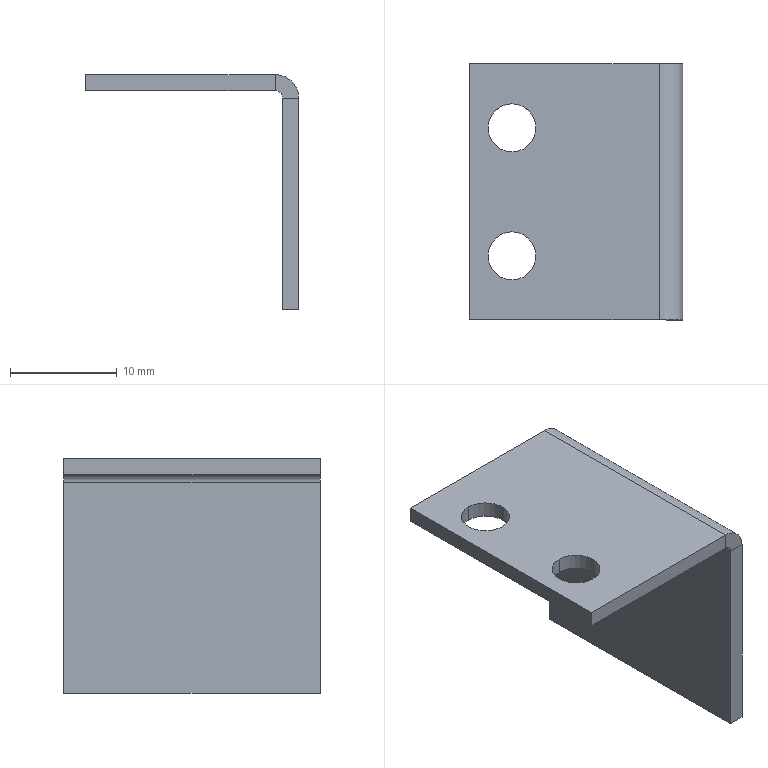Component | SolidWorks | 17081801-804-017B-1 | 1 solid | 18 faces | box 20 x 24 x 22 mm | volume 1388 mm3 | plane 12 | cylinder 6 | commonest cylinder face diameters 4.5 x4 4.4 x1 1.4 x1 | material 1.5mm304 Stainless Steel
STEP:
#1=COLOUR_RGB('',0.7922,0.8196,0.9333);
#2=FILL_AREA_STYLE_COLOUR('',#1);
#3=FILL_AREA_STYLE('',(#2));
#4=SURFACE_STYLE_FILL_AREA(#3);
#5=SURFACE_SIDE_STYLE('',(#4));
#6=SURFACE_STYLE_USAGE(.BOTH.,#5);
#7=PRESENTATION_STYLE_ASSIGNMENT((#6));
#8=CARTESIAN_POINT('',(1.043,83.234,5.335));
#9=VERTEX_POINT('',#8);
#10=CARTESIAN_POINT('',(1.043,83.057,5.335));
#11=VERTEX_POINT('',#10);
#12=CARTESIAN_POINT('',(1.043,83.146,5.335));
#13=DIRECTION('',(0.,-0.,1.));
#14=DIRECTION('',(-0.,-1.,0.));
#15=AXIS2_PLACEMENT_3D('',#12,#13,#14);
#16=CIRCLE('',#15,0.08858);
#17=EDGE_CURVE('',#9,#11,#16,.T.);
#18=ORIENTED_EDGE('',*,*,#17,.T.);
#19=CARTESIAN_POINT('',(1.043,83.057,5.276));
#20=VERTEX_POINT('',#19);
#21=CARTESIAN_POINT('',(1.043,83.057,5.276));
#22=DIRECTION('',(-0.,0.,-1.));
#23=VECTOR('',#22,39.37);
#24=LINE('',#21,#23);
#25=EDGE_CURVE('',#11,#20,#24,.T.);
#26=ORIENTED_EDGE('',*,*,#25,.T.);
#27=CARTESIAN_POINT('',(1.043,83.234,5.276));
#28=VERTEX_POINT('',#27);
#29=CARTESIAN_POINT('',(1.043,83.146,5.276));
#30=DIRECTION('',(-0.,0.,-1.));
#31=DIRECTION('',(0.,1.,0.));
#32=AXIS2_PLACEMENT_3D('',#29,#30,#31);
#33=CIRCLE('',#32,0.08858);
#34=EDGE_CURVE('',#20,#28,#33,.T.);
#35=ORIENTED_EDGE('',*,*,#34,.T.);
#36=CARTESIAN_POINT('',(1.043,83.234,5.276));
#37=DIRECTION('',(-0.,0.,-1.));
#38=VECTOR('',#37,39.37);
#39=LINE('',#36,#38);
#40=EDGE_CURVE('',#9,#28,#39,.T.);
#41=ORIENTED_EDGE('',*,*,#40,.F.);
#42=EDGE_LOOP('',(#18,#26,#35,#41));
#43=FACE_OUTER_BOUND('',#42,.T.);
#44=CARTESIAN_POINT('',(1.043,83.146,5.276));
#45=DIRECTION('',(-0.,0.,-1.));
#46=DIRECTION('',(0.,1.,0.));
#47=AXIS2_PLACEMENT_3D('',#44,#45,#46);
#48=CYLINDRICAL_SURFACE('',#47,0.08858);
#49=ADVANCED_FACE('',(#43),#48,.F.);
#50=CARTESIAN_POINT('',(1.043,83.707,5.335));
#51=VERTEX_POINT('',#50);
#52=CARTESIAN_POINT('',(1.043,83.53,5.335));
#53=VERTEX_POINT('',#52);
#54=CARTESIAN_POINT('',(1.043,83.618,5.335));
#55=DIRECTION('',(0.,-0.,1.));
#56=DIRECTION('',(-0.,-1.,0.));
#57=AXIS2_PLACEMENT_3D('',#54,#55,#56);
#58=CIRCLE('',#57,0.08858);
#59=EDGE_CURVE('',#51,#53,#58,.T.);
#60=ORIENTED_EDGE('',*,*,#59,.T.);
#61=CARTESIAN_POINT('',(1.043,83.53,5.276));
#62=VERTEX_POINT('',#61);
#63=CARTESIAN_POINT('',(1.043,83.53,5.276));
#64=DIRECTION('',(-0.,0.,-1.));
#65=VECTOR('',#64,39.37);
#66=LINE('',#63,#65);
#67=EDGE_CURVE('',#53,#62,#66,.T.);
#68=ORIENTED_EDGE('',*,*,#67,.T.);
#69=CARTESIAN_POINT('',(1.043,83.707,5.276));
#70=VERTEX_POINT('',#69);
#71=CARTESIAN_POINT('',(1.043,83.618,5.276));
#72=DIRECTION('',(-0.,0.,-1.));
#73=DIRECTION('',(0.,1.,0.));
#74=AXIS2_PLACEMENT_3D('',#71,#72,#73);
#75=CIRCLE('',#74,0.08858);
#76=EDGE_CURVE('',#62,#70,#75,.T.);
#77=ORIENTED_EDGE('',*,*,#76,.T.);
#78=CARTESIAN_POINT('',(1.043,83.707,5.276));
#79=DIRECTION('',(-0.,0.,-1.));
#80=VECTOR('',#79,39.37);
#81=LINE('',#78,#80);
#82=EDGE_CURVE('',#51,#70,#81,.T.);
#83=ORIENTED_EDGE('',*,*,#82,.F.);
#84=EDGE_LOOP('',(#60,#68,#77,#83));
#85=FACE_OUTER_BOUND('',#84,.T.);
#86=CARTESIAN_POINT('',(1.043,83.618,5.276));
#87=DIRECTION('',(-0.,0.,-1.));
#88=DIRECTION('',(0.,1.,0.));
#89=AXIS2_PLACEMENT_3D('',#86,#87,#88);
#90=CYLINDRICAL_SURFACE('',#89,0.08858);
#91=ADVANCED_FACE('',(#85),#90,.F.);
#92=CARTESIAN_POINT('',(1.673,82.909,5.248));
#93=VERTEX_POINT('',#92);
#94=CARTESIAN_POINT('',(1.614,82.909,5.248));
#95=VERTEX_POINT('',#94);
#96=CARTESIAN_POINT('',(1.673,82.909,5.248));
#97=DIRECTION('',(-1.,0.,0.));
#98=VECTOR('',#97,39.37);
#99=LINE('',#96,#98);
#100=EDGE_CURVE('',#93,#95,#99,.T.);
#101=ORIENTED_EDGE('',*,*,#100,.F.);
#102=CARTESIAN_POINT('',(1.587,82.909,5.335));
#103=VERTEX_POINT('',#102);
#104=CARTESIAN_POINT('',(1.587,82.909,5.248));
#105=DIRECTION('',(0.,1.,0.));
#106=DIRECTION('',(1.,0.,0.));
#107=AXIS2_PLACEMENT_3D('',#104,#105,#106);
#108=CIRCLE('',#107,0.08661);
#109=EDGE_CURVE('',#103,#93,#108,.T.);
#110=ORIENTED_EDGE('',*,*,#109,.F.);
#111=CARTESIAN_POINT('',(1.587,82.909,5.276));
#112=VERTEX_POINT('',#111);
#113=CARTESIAN_POINT('',(1.587,82.909,5.276));
#114=DIRECTION('',(-0.,-0.,1.));
#115=VECTOR('',#114,39.37);
#116=LINE('',#113,#115);
#117=EDGE_CURVE('',#112,#103,#116,.T.);
#118=ORIENTED_EDGE('',*,*,#117,.F.);
#119=CARTESIAN_POINT('',(1.587,82.909,5.248));
#120=DIRECTION('',(0.,1.,0.));
#121=DIRECTION('',(1.,0.,0.));
#122=AXIS2_PLACEMENT_3D('',#119,#120,#121);
#123=CIRCLE('',#122,0.02756);
#124=EDGE_CURVE('',#112,#95,#123,.T.);
#125=ORIENTED_EDGE('',*,*,#124,.T.);
#126=EDGE_LOOP('',(#101,#110,#118,#125));
#127=FACE_OUTER_BOUND('',#126,.T.);
#128=CARTESIAN_POINT('',(1.673,82.909,5.248));
#129=DIRECTION('',(-0.,-1.,-0.));
#130=DIRECTION('',(1.,-0.,-0.));
#131=AXIS2_PLACEMENT_3D('',#128,#129,#130);
#132=PLANE('',#131);
#133=ADVANCED_FACE('',(#127),#132,.T.);
#134=CARTESIAN_POINT('',(1.673,82.909,4.469));
#135=VERTEX_POINT('',#134);
#136=CARTESIAN_POINT('',(1.673,82.909,5.335));
#137=DIRECTION('',(0.,0.,-1.));
#138=VECTOR('',#137,39.37);
#139=LINE('',#136,#138);
#140=EDGE_CURVE('',#93,#135,#139,.T.);
#141=ORIENTED_EDGE('',*,*,#140,.F.);
#142=ORIENTED_EDGE('',*,*,#100,.T.);
#143=CARTESIAN_POINT('',(1.614,82.909,4.469));
#144=VERTEX_POINT('',#143);
#145=CARTESIAN_POINT('',(1.614,82.909,5.335));
#146=DIRECTION('',(0.,0.,-1.));
#147=VECTOR('',#146,39.37);
#148=LINE('',#145,#147);
#149=EDGE_CURVE('',#95,#144,#148,.T.);
#150=ORIENTED_EDGE('',*,*,#149,.T.);
#151=CARTESIAN_POINT('',(1.673,82.909,4.469));
#152=DIRECTION('',(-1.,0.,0.));
#153=VECTOR('',#152,39.37);
#154=LINE('',#151,#153);
#155=EDGE_CURVE('',#135,#144,#154,.T.);
#156=ORIENTED_EDGE('',*,*,#155,.F.);
#157=EDGE_LOOP('',(#141,#142,#150,#156));
#158=FACE_OUTER_BOUND('',#157,.T.);
#159=CARTESIAN_POINT('',(1.587,82.909,5.276));
#160=DIRECTION('',(-0.,-1.,-0.));
#161=DIRECTION('',(1.,-0.,-0.));
#162=AXIS2_PLACEMENT_3D('',#159,#160,#161);
#163=PLANE('',#162);
#164=ADVANCED_FACE('',(#158),#163,.T.);
#165=CARTESIAN_POINT('',(1.587,83.854,5.335));
#166=VERTEX_POINT('',#165);
#167=CARTESIAN_POINT('',(1.587,83.854,5.276));
#168=VERTEX_POINT('',#167);
#169=CARTESIAN_POINT('',(1.587,83.854,5.335));
#170=DIRECTION('',(0.,0.,-1.));
#171=VECTOR('',#170,39.37);
#172=LINE('',#169,#171);
#173=EDGE_CURVE('',#166,#168,#172,.T.);
#174=ORIENTED_EDGE('',*,*,#173,.F.);
#175=CARTESIAN_POINT('',(1.673,83.854,5.248));
#176=VERTEX_POINT('',#175);
#177=CARTESIAN_POINT('',(1.587,83.854,5.248));
#178=DIRECTION('',(0.,1.,0.));
#179=DIRECTION('',(1.,0.,0.));
#180=AXIS2_PLACEMENT_3D('',#177,#178,#179);
#181=CIRCLE('',#180,0.08661);
#182=EDGE_CURVE('',#166,#176,#181,.T.);
#183=ORIENTED_EDGE('',*,*,#182,.T.);
#184=CARTESIAN_POINT('',(1.614,83.854,5.248));
#185=VERTEX_POINT('',#184);
#186=CARTESIAN_POINT('',(1.614,83.854,5.248));
#187=DIRECTION('',(1.,-0.,-0.));
#188=VECTOR('',#187,39.37);
#189=LINE('',#186,#188);
#190=EDGE_CURVE('',#185,#176,#189,.T.);
#191=ORIENTED_EDGE('',*,*,#190,.F.);
#192=CARTESIAN_POINT('',(1.587,83.854,5.248));
#193=DIRECTION('',(0.,1.,0.));
#194=DIRECTION('',(1.,0.,0.));
#195=AXIS2_PLACEMENT_3D('',#192,#193,#194);
#196=CIRCLE('',#195,0.02756);
#197=EDGE_CURVE('',#168,#185,#196,.T.);
#198=ORIENTED_EDGE('',*,*,#197,.F.);
#199=EDGE_LOOP('',(#174,#183,#191,#198));
#200=FACE_OUTER_BOUND('',#199,.T.);
#201=CARTESIAN_POINT('',(1.587,83.854,5.335));
#202=DIRECTION('',(0.,1.,0.));
#203=DIRECTION('',(-1.,0.,0.));
#204=AXIS2_PLACEMENT_3D('',#201,#202,#203);
#205=PLANE('',#204);
#206=ADVANCED_FACE('',(#200),#205,.T.);
#207=CARTESIAN_POINT('',(0.8858,83.854,5.335));
#208=VERTEX_POINT('',#207);
#209=CARTESIAN_POINT('',(0.8858,83.854,5.335));
#210=DIRECTION('',(1.,-0.,-0.));
#211=VECTOR('',#210,39.37);
#212=LINE('',#209,#211);
#213=EDGE_CURVE('',#208,#166,#212,.T.);
#214=ORIENTED_EDGE('',*,*,#213,.T.);
#215=ORIENTED_EDGE('',*,*,#173,.T.);
#216=CARTESIAN_POINT('',(0.8858,83.854,5.276));
#217=VERTEX_POINT('',#216);
#218=CARTESIAN_POINT('',(0.8858,83.854,5.276));
#219=DIRECTION('',(1.,-0.,-0.));
#220=VECTOR('',#219,39.37);
#221=LINE('',#218,#220);
#222=EDGE_CURVE('',#217,#168,#221,.T.);
#223=ORIENTED_EDGE('',*,*,#222,.F.);
#224=CARTESIAN_POINT('',(0.8858,83.854,5.276));
#225=DIRECTION('',(0.,-0.,1.));
#226=VECTOR('',#225,39.37);
#227=LINE('',#224,#226);
#228=EDGE_CURVE('',#217,#208,#227,.T.);
#229=ORIENTED_EDGE('',*,*,#228,.T.);
#230=EDGE_LOOP('',(#214,#215,#223,#229));
#231=FACE_OUTER_BOUND('',#230,.T.);
#232=CARTESIAN_POINT('',(1.614,83.854,5.248));
#233=DIRECTION('',(0.,1.,0.));
#234=DIRECTION('',(-1.,0.,0.));
#235=AXIS2_PLACEMENT_3D('',#232,#233,#234);
#236=PLANE('',#235);
#237=ADVANCED_FACE('',(#231),#236,.T.);
#238=CARTESIAN_POINT('',(1.614,83.854,4.469));
#239=VERTEX_POINT('',#238);
#240=CARTESIAN_POINT('',(1.614,83.854,5.335));
#241=DIRECTION('',(0.,0.,-1.));
#242=VECTOR('',#241,39.37);
#243=LINE('',#240,#242);
#244=EDGE_CURVE('',#185,#239,#243,.T.);
#245=ORIENTED_EDGE('',*,*,#244,.T.);
#246=CARTESIAN_POINT('',(1.614,82.909,4.469));
#247=DIRECTION('',(0.,1.,0.));
#248=VECTOR('',#247,39.37);
#249=LINE('',#246,#248);
#250=EDGE_CURVE('',#144,#239,#249,.T.);
#251=ORIENTED_EDGE('',*,*,#250,.F.);
#252=ORIENTED_EDGE('',*,*,#149,.F.);
#253=CARTESIAN_POINT('',(1.614,82.909,5.248));
#254=DIRECTION('',(0.,1.,0.));
#255=VECTOR('',#254,39.37);
#256=LINE('',#253,#255);
#257=EDGE_CURVE('',#95,#185,#256,.T.);
#258=ORIENTED_EDGE('',*,*,#257,.T.);
#259=EDGE_LOOP('',(#245,#251,#252,#258));
#260=FACE_OUTER_BOUND('',#259,.T.);
#261=CARTESIAN_POINT('',(1.614,82.909,5.335));
#262=DIRECTION('',(1.,-0.,0.));
#263=DIRECTION('',(-0.,-0.,1.));
#264=AXIS2_PLACEMENT_3D('',#261,#262,#263);
#265=PLANE('',#264);
#266=ADVANCED_FACE('',(#260),#265,.F.);
#267=CARTESIAN_POINT('',(1.673,83.854,4.469));
#268=VERTEX_POINT('',#267);
#269=CARTESIAN_POINT('',(1.673,83.854,4.469));
#270=DIRECTION('',(-1.,0.,0.));
#271=VECTOR('',#270,39.37);
#272=LINE('',#269,#271);
#273=EDGE_CURVE('',#268,#239,#272,.T.);
#274=ORIENTED_EDGE('',*,*,#273,.F.);
#275=CARTESIAN_POINT('',(1.673,82.909,4.469));
#276=DIRECTION('',(0.,1.,0.));
#277=VECTOR('',#276,39.37);
#278=LINE('',#275,#277);
#279=EDGE_CURVE('',#135,#268,#278,.T.);
#280=ORIENTED_EDGE('',*,*,#279,.F.);
#281=ORIENTED_EDGE('',*,*,#155,.T.);
#282=ORIENTED_EDGE('',*,*,#250,.T.);
#283=EDGE_LOOP('',(#274,#280,#281,#282));
#284=FACE_OUTER_BOUND('',#283,.T.);
#285=CARTESIAN_POINT('',(1.673,82.909,4.469));
#286=DIRECTION('',(-0.,0.,-1.));
#287=DIRECTION('',(0.,1.,0.));
#288=AXIS2_PLACEMENT_3D('',#285,#286,#287);
#289=PLANE('',#288);
#290=ADVANCED_FACE('',(#284),#289,.T.);
#291=CARTESIAN_POINT('',(1.673,83.854,5.335));
#292=DIRECTION('',(0.,0.,-1.));
#293=VECTOR('',#292,39.37);
#294=LINE('',#291,#293);
#295=EDGE_CURVE('',#176,#268,#294,.T.);
#296=ORIENTED_EDGE('',*,*,#295,.F.);
#297=CARTESIAN_POINT('',(1.673,82.909,5.248));
#298=DIRECTION('',(0.,1.,0.));
#299=VECTOR('',#298,39.37);
#300=LINE('',#297,#299);
#301=EDGE_CURVE('',#93,#176,#300,.T.);
#302=ORIENTED_EDGE('',*,*,#301,.F.);
#303=ORIENTED_EDGE('',*,*,#140,.T.);
#304=ORIENTED_EDGE('',*,*,#279,.T.);
#305=EDGE_LOOP('',(#296,#302,#303,#304));
#306=FACE_OUTER_BOUND('',#305,.T.);
#307=CARTESIAN_POINT('',(1.673,82.909,5.335));
#308=DIRECTION('',(1.,-0.,0.));
#309=DIRECTION('',(-0.,-0.,1.));
#310=AXIS2_PLACEMENT_3D('',#307,#308,#309);
#311=PLANE('',#310);
#312=ADVANCED_FACE('',(#306),#311,.T.);
#313=ORIENTED_EDGE('',*,*,#182,.F.);
#314=CARTESIAN_POINT('',(1.587,82.909,5.335));
#315=DIRECTION('',(0.,1.,0.));
#316=VECTOR('',#315,39.37);
#317=LINE('',#314,#316);
#318=EDGE_CURVE('',#103,#166,#317,.T.);
#319=ORIENTED_EDGE('',*,*,#318,.F.);
#320=ORIENTED_EDGE('',*,*,#109,.T.);
#321=ORIENTED_EDGE('',*,*,#301,.T.);
#322=EDGE_LOOP('',(#313,#319,#320,#321));
#323=FACE_OUTER_BOUND('',#322,.T.);
#324=CARTESIAN_POINT('',(1.587,82.909,5.248));
#325=DIRECTION('',(0.,1.,0.));
#326=DIRECTION('',(-1.,0.,0.));
#327=AXIS2_PLACEMENT_3D('',#324,#325,#326);
#328=CYLINDRICAL_SURFACE('',#327,0.08661);
#329=ADVANCED_FACE('',(#323),#328,.T.);
#330=ORIENTED_EDGE('',*,*,#17,.F.);
#331=CARTESIAN_POINT('',(1.043,83.146,5.335));
#332=DIRECTION('',(0.,-0.,1.));
#333=DIRECTION('',(-0.,-1.,0.));
#334=AXIS2_PLACEMENT_3D('',#331,#332,#333);
#335=CIRCLE('',#334,0.08858);
#336=EDGE_CURVE('',#11,#9,#335,.T.);
#337=ORIENTED_EDGE('',*,*,#336,.F.);
#338=EDGE_LOOP('',(#330,#337));
#339=FACE_BOUND('',#338,.T.);
#340=ORIENTED_EDGE('',*,*,#59,.F.);
#341=CARTESIAN_POINT('',(1.043,83.618,5.335));
#342=DIRECTION('',(0.,-0.,1.));
#343=DIRECTION('',(-0.,-1.,0.));
#344=AXIS2_PLACEMENT_3D('',#341,#342,#343);
#345=CIRCLE('',#344,0.08858);
#346=EDGE_CURVE('',#53,#51,#345,.T.);
#347=ORIENTED_EDGE('',*,*,#346,.F.);
#348=EDGE_LOOP('',(#340,#347));
#349=FACE_BOUND('',#348,.T.);
#350=ORIENTED_EDGE('',*,*,#213,.F.);
#351=CARTESIAN_POINT('',(0.8858,82.909,5.335));
#352=VERTEX_POINT('',#351);
#353=CARTESIAN_POINT('',(0.8858,82.909,5.335));
#354=DIRECTION('',(0.,1.,0.));
#355=VECTOR('',#354,39.37);
#356=LINE('',#353,#355);
#357=EDGE_CURVE('',#352,#208,#356,.T.);
#358=ORIENTED_EDGE('',*,*,#357,.F.);
#359=CARTESIAN_POINT('',(0.8858,82.909,5.335));
#360=DIRECTION('',(1.,-0.,-0.));
#361=VECTOR('',#360,39.37);
#362=LINE('',#359,#361);
#363=EDGE_CURVE('',#352,#103,#362,.T.);
#364=ORIENTED_EDGE('',*,*,#363,.T.);
#365=ORIENTED_EDGE('',*,*,#318,.T.);
#366=EDGE_LOOP('',(#350,#358,#364,#365));
#367=FACE_OUTER_BOUND('',#366,.T.);
#368=CARTESIAN_POINT('',(0.8858,82.909,5.335));
#369=DIRECTION('',(0.,-0.,1.));
#370=DIRECTION('',(-0.,-1.,-0.));
#371=AXIS2_PLACEMENT_3D('',#368,#369,#370);
#372=PLANE('',#371);
#373=ADVANCED_FACE('',(#339,#349,#367),#372,.T.);
#374=ORIENTED_EDGE('',*,*,#228,.F.);
#375=CARTESIAN_POINT('',(0.8858,82.909,5.276));
#376=VERTEX_POINT('',#375);
#377=CARTESIAN_POINT('',(0.8858,82.909,5.276));
#378=DIRECTION('',(0.,1.,0.));
#379=VECTOR('',#378,39.37);
#380=LINE('',#377,#379);
#381=EDGE_CURVE('',#376,#217,#380,.T.);
#382=ORIENTED_EDGE('',*,*,#381,.F.);
#383=CARTESIAN_POINT('',(0.8858,82.909,5.276));
#384=DIRECTION('',(0.,-0.,1.));
#385=VECTOR('',#384,39.37);
#386=LINE('',#383,#385);
#387=EDGE_CURVE('',#376,#352,#386,.T.);
#388=ORIENTED_EDGE('',*,*,#387,.T.);
#389=ORIENTED_EDGE('',*,*,#357,.T.);
#390=EDGE_LOOP('',(#374,#382,#388,#389));
#391=FACE_OUTER_BOUND('',#390,.T.);
#392=CARTESIAN_POINT('',(0.8858,82.909,5.276));
#393=DIRECTION('',(-1.,0.,0.));
#394=DIRECTION('',(-0.,-1.,-0.));
#395=AXIS2_PLACEMENT_3D('',#392,#393,#394);
#396=PLANE('',#395);
#397=ADVANCED_FACE('',(#391),#396,.T.);
#398=CARTESIAN_POINT('',(1.043,83.146,5.276));
#399=DIRECTION('',(-0.,0.,-1.));
#400=DIRECTION('',(0.,1.,0.));
#401=AXIS2_PLACEMENT_3D('',#398,#399,#400);
#402=CIRCLE('',#401,0.08858);
#403=EDGE_CURVE('',#28,#20,#402,.T.);
#404=ORIENTED_EDGE('',*,*,#403,.F.);
#405=ORIENTED_EDGE('',*,*,#34,.F.);
#406=EDGE_LOOP('',(#404,#405));
#407=FACE_BOUND('',#406,.T.);
#408=CARTESIAN_POINT('',(1.043,83.618,5.276));
#409=DIRECTION('',(-0.,0.,-1.));
#410=DIRECTION('',(0.,1.,0.));
#411=AXIS2_PLACEMENT_3D('',#408,#409,#410);
#412=CIRCLE('',#411,0.08858);
#413=EDGE_CURVE('',#70,#62,#412,.T.);
#414=ORIENTED_EDGE('',*,*,#413,.F.);
#415=ORIENTED_EDGE('',*,*,#76,.F.);
#416=EDGE_LOOP('',(#414,#415));
#417=FACE_BOUND('',#416,.T.);
#418=ORIENTED_EDGE('',*,*,#222,.T.);
#419=CARTESIAN_POINT('',(1.587,82.909,5.276));
#420=DIRECTION('',(0.,1.,0.));
#421=VECTOR('',#420,39.37);
#422=LINE('',#419,#421);
#423=EDGE_CURVE('',#112,#168,#422,.T.);
#424=ORIENTED_EDGE('',*,*,#423,.F.);
#425=CARTESIAN_POINT('',(0.8858,82.909,5.276));
#426=DIRECTION('',(1.,-0.,-0.));
#427=VECTOR('',#426,39.37);
#428=LINE('',#425,#427);
#429=EDGE_CURVE('',#376,#112,#428,.T.);
#430=ORIENTED_EDGE('',*,*,#429,.F.);
#431=ORIENTED_EDGE('',*,*,#381,.T.);
#432=EDGE_LOOP('',(#418,#424,#430,#431));
#433=FACE_OUTER_BOUND('',#432,.T.);
#434=CARTESIAN_POINT('',(0.8858,82.909,5.276));
#435=DIRECTION('',(0.,-0.,1.));
#436=DIRECTION('',(-0.,-1.,-0.));
#437=AXIS2_PLACEMENT_3D('',#434,#435,#436);
#438=PLANE('',#437);
#439=ADVANCED_FACE('',(#407,#417,#433),#438,.F.);
#440=ORIENTED_EDGE('',*,*,#197,.T.);
#441=ORIENTED_EDGE('',*,*,#257,.F.);
#442=ORIENTED_EDGE('',*,*,#124,.F.);
#443=ORIENTED_EDGE('',*,*,#423,.T.);
#444=EDGE_LOOP('',(#440,#441,#442,#443));
#445=FACE_OUTER_BOUND('',#444,.T.);
#446=CARTESIAN_POINT('',(1.587,82.909,5.248));
#447=DIRECTION('',(0.,1.,0.));
#448=DIRECTION('',(-1.,0.,0.));
#449=AXIS2_PLACEMENT_3D('',#446,#447,#448);
#450=CYLINDRICAL_SURFACE('',#449,0.02756);
#451=ADVANCED_FACE('',(#445),#450,.F.);
#452=ORIENTED_EDGE('',*,*,#429,.T.);
#453=ORIENTED_EDGE('',*,*,#117,.T.);
#454=ORIENTED_EDGE('',*,*,#363,.F.);
#455=ORIENTED_EDGE('',*,*,#387,.F.);
#456=EDGE_LOOP('',(#452,#453,#454,#455));
#457=FACE_OUTER_BOUND('',#456,.T.);
#458=CARTESIAN_POINT('',(1.587,82.909,5.248));
#459=DIRECTION('',(-0.,-1.,-0.));
#460=DIRECTION('',(1.,-0.,-0.));
#461=AXIS2_PLACEMENT_3D('',#458,#459,#460);
#462=PLANE('',#461);
#463=ADVANCED_FACE('',(#457),#462,.T.);
#464=ORIENTED_EDGE('',*,*,#244,.F.);
#465=ORIENTED_EDGE('',*,*,#190,.T.);
#466=ORIENTED_EDGE('',*,*,#295,.T.);
#467=ORIENTED_EDGE('',*,*,#273,.T.);
#468=EDGE_LOOP('',(#464,#465,#466,#467));
#469=FACE_OUTER_BOUND('',#468,.T.);
#470=CARTESIAN_POINT('',(1.587,83.854,5.248));
#471=DIRECTION('',(-0.,-1.,-0.));
#472=DIRECTION('',(1.,-0.,-0.));
#473=AXIS2_PLACEMENT_3D('',#470,#471,#472);
#474=PLANE('',#473);
#475=ADVANCED_FACE('',(#469),#474,.F.);
#476=ORIENTED_EDGE('',*,*,#67,.F.);
#477=ORIENTED_EDGE('',*,*,#346,.T.);
#478=ORIENTED_EDGE('',*,*,#82,.T.);
#479=ORIENTED_EDGE('',*,*,#413,.T.);
#480=EDGE_LOOP('',(#476,#477,#478,#479));
#481=FACE_OUTER_BOUND('',#480,.T.);
#482=CARTESIAN_POINT('',(1.043,83.618,5.276));
#483=DIRECTION('',(-0.,0.,-1.));
#484=DIRECTION('',(0.,1.,0.));
#485=AXIS2_PLACEMENT_3D('',#482,#483,#484);
#486=CYLINDRICAL_SURFACE('',#485,0.08858);
#487=ADVANCED_FACE('',(#481),#486,.F.);
#488=ORIENTED_EDGE('',*,*,#25,.F.);
#489=ORIENTED_EDGE('',*,*,#336,.T.);
#490=ORIENTED_EDGE('',*,*,#40,.T.);
#491=ORIENTED_EDGE('',*,*,#403,.T.);
#492=EDGE_LOOP('',(#488,#489,#490,#491));
#493=FACE_OUTER_BOUND('',#492,.T.);
#494=CARTESIAN_POINT('',(1.043,83.146,5.276));
#495=DIRECTION('',(-0.,0.,-1.));
#496=DIRECTION('',(0.,1.,0.));
#497=AXIS2_PLACEMENT_3D('',#494,#495,#496);
#498=CYLINDRICAL_SURFACE('',#497,0.08858);
#499=ADVANCED_FACE('',(#493),#498,.F.);
#500=CLOSED_SHELL('',(#49,#91,#133,#164,#206,#237,#266,#290,#312,#329,#373,#397,#439,#451,#463,#475,#487,#499));
#501=MANIFOLD_SOLID_BREP('',#500);
#502=STYLED_ITEM('',(#7),#501);
#503=(LENGTH_UNIT()NAMED_UNIT(*)SI_UNIT($,.METRE.));
#504=LENGTH_MEASURE_WITH_UNIT(LENGTH_MEASURE(0.0254),#503);
#505=DIMENSIONAL_EXPONENTS(1.,0.,0.,0.,0.,0.,0.);
#506=(CONVERSION_BASED_UNIT('',#504)LENGTH_UNIT()NAMED_UNIT(#505));
#507=UNCERTAINTY_MEASURE_WITH_UNIT(LENGTH_MEASURE(0.00001),#506,'','');
#508=(NAMED_UNIT(*)PLANE_ANGLE_UNIT()SI_UNIT($,.RADIAN.));
#509=(NAMED_UNIT(*)SI_UNIT($,.STERADIAN.)SOLID_ANGLE_UNIT());
#510=(GEOMETRIC_REPRESENTATION_CONTEXT(3)GLOBAL_UNCERTAINTY_ASSIGNED_CONTEXT((#507))GLOBAL_UNIT_ASSIGNED_CONTEXT((#506,#508,#509))REPRESENTATION_CONTEXT('',''));
#511=MECHANICAL_DESIGN_GEOMETRIC_PRESENTATION_REPRESENTATION('',(#502),#510);
#512=CARTESIAN_POINT('',(0.,0.,0.));
#513=DIRECTION('',(0.,0.,1.));
#514=DIRECTION('',(1.,0.,0.));
#515=AXIS2_PLACEMENT_3D('',#512,#513,#514);
#516=(LENGTH_UNIT()NAMED_UNIT(*)SI_UNIT($,.METRE.));
#517=LENGTH_MEASURE_WITH_UNIT(LENGTH_MEASURE(0.0254),#516);
#518=DIMENSIONAL_EXPONENTS(1.,0.,0.,0.,0.,0.,0.);
#519=(CONVERSION_BASED_UNIT('',#517)LENGTH_UNIT()NAMED_UNIT(#518));
#520=UNCERTAINTY_MEASURE_WITH_UNIT(LENGTH_MEASURE(0.00001),#519,'','');
#521=(NAMED_UNIT(*)PLANE_ANGLE_UNIT()SI_UNIT($,.RADIAN.));
#522=(NAMED_UNIT(*)SI_UNIT($,.STERADIAN.)SOLID_ANGLE_UNIT());
#523=(GEOMETRIC_REPRESENTATION_CONTEXT(3)GLOBAL_UNCERTAINTY_ASSIGNED_CONTEXT((#520))GLOBAL_UNIT_ASSIGNED_CONTEXT((#519,#521,#522))REPRESENTATION_CONTEXT('',''));
#524=ADVANCED_BREP_SHAPE_REPRESENTATION('',(#501,#515),#523);
#525=PRESENTATION_LAYER_ASSIGNMENT('','',(#502));